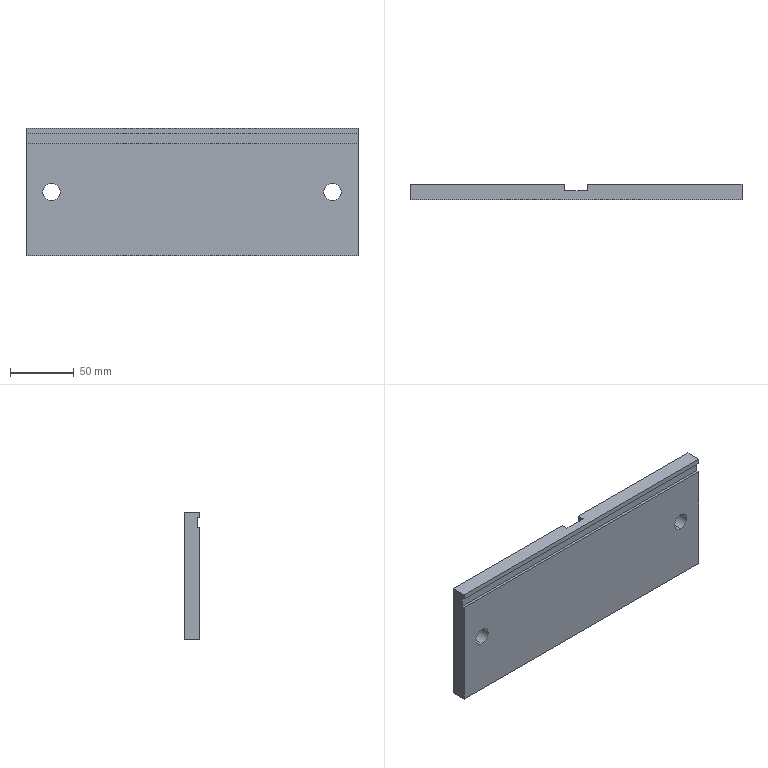Component | SolidWorks | NewTypeCurveBenderReducerPlate-DoubleWheel-2_NewCurveBender(New)ReducerBasePlate-DoubleWheel-1 | 1 solid | 18 faces | box 260 x 12 x 100 mm | volume 295405 mm3 | plane 14 | cylinder 4 | commonest cylinder face diameters 13.5 x4
build123d program:
from build123d import *

# Parameters (mm, degrees)
SKETCH1_W           = 260
SKETCH1_H           = 100
BOSS_EXTRUDE1_DEPTH = 12
SKETCH2_W           = 18
SKETCH2_H           = 5
CUT_EXTRUDE1_DEPTH  = 165.451
SKETCH3_R           = 6.75
CUT_EXTRUDE2_DEPTH  = 12
SKETCH5_W           = 8
SKETCH5_H           = 2
CUT_EXTRUDE3_DEPTH  = 266.036


with BuildPart() as part:
    # Sketch1 → Boss-Extrude1 (new body)
    with BuildSketch(Plane(origin=(0, 0, 0), x_dir=(1, 0, 0), z_dir=(0, 1, 0))):
        Rectangle(SKETCH1_W, SKETCH1_H)
    extrude(amount=BOSS_EXTRUDE1_DEPTH)

    # Sketch2 → Cut-Extrude1 (cut, through all)
    with BuildSketch(Plane.XY.offset(50)):
        with Locations((0, 2.5)):
            Rectangle(SKETCH2_W, SKETCH2_H)
    extrude(amount=-CUT_EXTRUDE1_DEPTH, mode=Mode.SUBTRACT)

    # Sketch3 → Cut-Extrude2 (cut)
    with BuildSketch(Plane(origin=(0, 12, 0), x_dir=(1, 0, 0), z_dir=(0, 1, 0))):
        with Locations(Location((-110, 0, 0), (0, 0, 270))):
            Circle(SKETCH3_R)
        with Locations(Location((110, 0, 0), (0, 0, 90))):
            Circle(SKETCH3_R)
    extrude(amount=-CUT_EXTRUDE2_DEPTH, mode=Mode.SUBTRACT)

    # Sketch5 → Cut-Extrude3 (cut, through all)
    with BuildSketch(Plane.ZY.offset(130)):
        with Locations((42, 11)):
            Rectangle(SKETCH5_W, SKETCH5_H)
    extrude(amount=-CUT_EXTRUDE3_DEPTH, mode=Mode.SUBTRACT)


solid = part.part

# Placed as in the assembly
solid = solid.moved(Location((0, 20, 158), (0, 0, 180)))
STEP:
#1=COLOUR_RGB('',0.7922,0.8196,0.9333);
#2=FILL_AREA_STYLE_COLOUR('',#1);
#3=FILL_AREA_STYLE('',(#2));
#4=SURFACE_STYLE_FILL_AREA(#3);
#5=SURFACE_SIDE_STYLE('',(#4));
#6=SURFACE_STYLE_USAGE(.BOTH.,#5);
#7=PRESENTATION_STYLE_ASSIGNMENT((#6));
#8=CARTESIAN_POINT('',(-4.331,0.7874,5.955));
#9=VERTEX_POINT('',#8);
#10=CARTESIAN_POINT('',(-4.331,0.7874,6.486));
#11=VERTEX_POINT('',#10);
#12=CARTESIAN_POINT('',(-4.331,0.7874,6.22));
#13=DIRECTION('',(-0.,-1.,-0.));
#14=DIRECTION('',(0.,0.,-1.));
#15=AXIS2_PLACEMENT_3D('',#12,#13,#14);
#16=CIRCLE('',#15,0.2657);
#17=EDGE_CURVE('',#9,#11,#16,.T.);
#18=ORIENTED_EDGE('',*,*,#17,.F.);
#19=CARTESIAN_POINT('',(-4.331,0.315,5.955));
#20=VERTEX_POINT('',#19);
#21=CARTESIAN_POINT('',(-4.331,0.7874,5.955));
#22=DIRECTION('',(-0.,-1.,-0.));
#23=VECTOR('',#22,39.37);
#24=LINE('',#21,#23);
#25=EDGE_CURVE('',#9,#20,#24,.T.);
#26=ORIENTED_EDGE('',*,*,#25,.T.);
#27=CARTESIAN_POINT('',(-4.331,0.315,6.486));
#28=VERTEX_POINT('',#27);
#29=CARTESIAN_POINT('',(-4.331,0.315,6.22));
#30=DIRECTION('',(-0.,-1.,-0.));
#31=DIRECTION('',(0.,0.,-1.));
#32=AXIS2_PLACEMENT_3D('',#29,#30,#31);
#33=CIRCLE('',#32,0.2657);
#34=EDGE_CURVE('',#20,#28,#33,.T.);
#35=ORIENTED_EDGE('',*,*,#34,.T.);
#36=CARTESIAN_POINT('',(-4.331,0.7874,6.486));
#37=DIRECTION('',(-0.,-1.,-0.));
#38=VECTOR('',#37,39.37);
#39=LINE('',#36,#38);
#40=EDGE_CURVE('',#11,#28,#39,.T.);
#41=ORIENTED_EDGE('',*,*,#40,.F.);
#42=EDGE_LOOP('',(#18,#26,#35,#41));
#43=FACE_OUTER_BOUND('',#42,.T.);
#44=CARTESIAN_POINT('',(-4.331,0.7874,6.22));
#45=DIRECTION('',(-0.,-1.,-0.));
#46=DIRECTION('',(0.,0.,1.));
#47=AXIS2_PLACEMENT_3D('',#44,#45,#46);
#48=CYLINDRICAL_SURFACE('',#47,0.2657);
#49=ADVANCED_FACE('',(#43),#48,.F.);
#50=CARTESIAN_POINT('',(4.331,0.7874,5.955));
#51=VERTEX_POINT('',#50);
#52=CARTESIAN_POINT('',(4.331,0.7874,6.486));
#53=VERTEX_POINT('',#52);
#54=CARTESIAN_POINT('',(4.331,0.7874,6.22));
#55=DIRECTION('',(-0.,-1.,-0.));
#56=DIRECTION('',(0.,0.,1.));
#57=AXIS2_PLACEMENT_3D('',#54,#55,#56);
#58=CIRCLE('',#57,0.2657);
#59=EDGE_CURVE('',#51,#53,#58,.T.);
#60=ORIENTED_EDGE('',*,*,#59,.F.);
#61=CARTESIAN_POINT('',(4.331,0.315,5.955));
#62=VERTEX_POINT('',#61);
#63=CARTESIAN_POINT('',(4.331,0.7874,5.955));
#64=DIRECTION('',(-0.,-1.,-0.));
#65=VECTOR('',#64,39.37);
#66=LINE('',#63,#65);
#67=EDGE_CURVE('',#51,#62,#66,.T.);
#68=ORIENTED_EDGE('',*,*,#67,.T.);
#69=CARTESIAN_POINT('',(4.331,0.315,6.486));
#70=VERTEX_POINT('',#69);
#71=CARTESIAN_POINT('',(4.331,0.315,6.22));
#72=DIRECTION('',(-0.,-1.,-0.));
#73=DIRECTION('',(0.,-0.,1.));
#74=AXIS2_PLACEMENT_3D('',#71,#72,#73);
#75=CIRCLE('',#74,0.2657);
#76=EDGE_CURVE('',#62,#70,#75,.T.);
#77=ORIENTED_EDGE('',*,*,#76,.T.);
#78=CARTESIAN_POINT('',(4.331,0.7874,6.486));
#79=DIRECTION('',(-0.,-1.,-0.));
#80=VECTOR('',#79,39.37);
#81=LINE('',#78,#80);
#82=EDGE_CURVE('',#53,#70,#81,.T.);
#83=ORIENTED_EDGE('',*,*,#82,.F.);
#84=EDGE_LOOP('',(#60,#68,#77,#83));
#85=FACE_OUTER_BOUND('',#84,.T.);
#86=CARTESIAN_POINT('',(4.331,0.7874,6.22));
#87=DIRECTION('',(-0.,-1.,-0.));
#88=DIRECTION('',(0.,0.,1.));
#89=AXIS2_PLACEMENT_3D('',#86,#87,#88);
#90=CYLINDRICAL_SURFACE('',#89,0.2657);
#91=ADVANCED_FACE('',(#85),#90,.F.);
#92=CARTESIAN_POINT('',(-5.118,0.315,7.717));
#93=VERTEX_POINT('',#92);
#94=CARTESIAN_POINT('',(5.118,0.315,7.717));
#95=VERTEX_POINT('',#94);
#96=CARTESIAN_POINT('',(-5.118,0.315,7.717));
#97=DIRECTION('',(1.,-0.,0.));
#98=VECTOR('',#97,39.37);
#99=LINE('',#96,#98);
#100=EDGE_CURVE('',#93,#95,#99,.T.);
#101=ORIENTED_EDGE('',*,*,#100,.F.);
#102=CARTESIAN_POINT('',(-5.118,0.315,4.252));
#103=VERTEX_POINT('',#102);
#104=CARTESIAN_POINT('',(-5.118,0.315,4.252));
#105=DIRECTION('',(0.,0.,-1.));
#106=VECTOR('',#105,39.37);
#107=LINE('',#104,#106);
#108=EDGE_CURVE('',#93,#103,#107,.T.);
#109=ORIENTED_EDGE('',*,*,#108,.T.);
#110=CARTESIAN_POINT('',(5.118,0.315,4.252));
#111=VERTEX_POINT('',#110);
#112=CARTESIAN_POINT('',(5.118,0.315,4.252));
#113=DIRECTION('',(1.,-0.,0.));
#114=VECTOR('',#113,39.37);
#115=LINE('',#112,#114);
#116=EDGE_CURVE('',#103,#111,#115,.T.);
#117=ORIENTED_EDGE('',*,*,#116,.T.);
#118=CARTESIAN_POINT('',(5.118,0.315,4.252));
#119=DIRECTION('',(-0.,-0.,1.));
#120=VECTOR('',#119,39.37);
#121=LINE('',#118,#120);
#122=EDGE_CURVE('',#111,#95,#121,.T.);
#123=ORIENTED_EDGE('',*,*,#122,.T.);
#124=EDGE_LOOP('',(#101,#109,#117,#123));
#125=FACE_OUTER_BOUND('',#124,.T.);
#126=CARTESIAN_POINT('',(4.331,0.315,6.22));
#127=DIRECTION('',(-0.,-1.,-0.));
#128=DIRECTION('',(0.,-0.,1.));
#129=AXIS2_PLACEMENT_3D('',#126,#127,#128);
#130=CIRCLE('',#129,0.2657);
#131=EDGE_CURVE('',#70,#62,#130,.T.);
#132=ORIENTED_EDGE('',*,*,#131,.F.);
#133=ORIENTED_EDGE('',*,*,#76,.F.);
#134=EDGE_LOOP('',(#132,#133));
#135=FACE_BOUND('',#134,.T.);
#136=CARTESIAN_POINT('',(-4.331,0.315,6.22));
#137=DIRECTION('',(-0.,-1.,-0.));
#138=DIRECTION('',(0.,0.,-1.));
#139=AXIS2_PLACEMENT_3D('',#136,#137,#138);
#140=CIRCLE('',#139,0.2657);
#141=EDGE_CURVE('',#28,#20,#140,.T.);
#142=ORIENTED_EDGE('',*,*,#141,.F.);
#143=ORIENTED_EDGE('',*,*,#34,.F.);
#144=EDGE_LOOP('',(#142,#143));
#145=FACE_BOUND('',#144,.T.);
#146=CARTESIAN_POINT('',(0.,0.315,6.22));
#147=DIRECTION('',(-0.,-1.,-0.));
#148=DIRECTION('',(-0.,-0.,1.));
#149=AXIS2_PLACEMENT_3D('',#146,#147,#148);
#150=PLANE('',#149);
#151=ADVANCED_FACE('',(#125,#135,#145),#150,.T.);
#152=CARTESIAN_POINT('',(-4.331,0.7874,6.22));
#153=DIRECTION('',(-0.,-1.,-0.));
#154=DIRECTION('',(0.,0.,-1.));
#155=AXIS2_PLACEMENT_3D('',#152,#153,#154);
#156=CIRCLE('',#155,0.2657);
#157=EDGE_CURVE('',#11,#9,#156,.T.);
#158=ORIENTED_EDGE('',*,*,#157,.T.);
#159=ORIENTED_EDGE('',*,*,#17,.T.);
#160=EDGE_LOOP('',(#158,#159));
#161=FACE_BOUND('',#160,.T.);
#162=CARTESIAN_POINT('',(-0.3543,0.7874,8.189));
#163=VERTEX_POINT('',#162);
#164=CARTESIAN_POINT('',(-5.118,0.7874,8.189));
#165=VERTEX_POINT('',#164);
#166=CARTESIAN_POINT('',(5.118,0.7874,8.189));
#167=DIRECTION('',(-1.,0.,-0.));
#168=VECTOR('',#167,39.37);
#169=LINE('',#166,#168);
#170=EDGE_CURVE('',#163,#165,#169,.T.);
#171=ORIENTED_EDGE('',*,*,#170,.F.);
#172=CARTESIAN_POINT('',(-0.3543,0.7874,4.252));
#173=VERTEX_POINT('',#172);
#174=CARTESIAN_POINT('',(-0.3543,0.7874,4.252));
#175=DIRECTION('',(-0.,-0.,1.));
#176=VECTOR('',#175,39.37);
#177=LINE('',#174,#176);
#178=EDGE_CURVE('',#173,#163,#177,.T.);
#179=ORIENTED_EDGE('',*,*,#178,.F.);
#180=CARTESIAN_POINT('',(-5.118,0.7874,4.252));
#181=VERTEX_POINT('',#180);
#182=CARTESIAN_POINT('',(5.118,0.7874,4.252));
#183=DIRECTION('',(1.,-0.,0.));
#184=VECTOR('',#183,39.37);
#185=LINE('',#182,#184);
#186=EDGE_CURVE('',#181,#173,#185,.T.);
#187=ORIENTED_EDGE('',*,*,#186,.F.);
#188=CARTESIAN_POINT('',(-5.118,0.7874,4.252));
#189=DIRECTION('',(0.,0.,-1.));
#190=VECTOR('',#189,39.37);
#191=LINE('',#188,#190);
#192=EDGE_CURVE('',#165,#181,#191,.T.);
#193=ORIENTED_EDGE('',*,*,#192,.F.);
#194=EDGE_LOOP('',(#171,#179,#187,#193));
#195=FACE_OUTER_BOUND('',#194,.T.);
#196=CARTESIAN_POINT('',(0.,0.7874,6.22));
#197=DIRECTION('',(-0.,-1.,-0.));
#198=DIRECTION('',(-0.,-0.,1.));
#199=AXIS2_PLACEMENT_3D('',#196,#197,#198);
#200=PLANE('',#199);
#201=ADVANCED_FACE('',(#161,#195),#200,.F.);
#202=ORIENTED_EDGE('',*,*,#108,.F.);
#203=CARTESIAN_POINT('',(-5.118,0.3937,7.717));
#204=VERTEX_POINT('',#203);
#205=CARTESIAN_POINT('',(-5.118,0.315,7.717));
#206=DIRECTION('',(0.,1.,0.));
#207=VECTOR('',#206,39.37);
#208=LINE('',#205,#207);
#209=EDGE_CURVE('',#93,#204,#208,.T.);
#210=ORIENTED_EDGE('',*,*,#209,.T.);
#211=CARTESIAN_POINT('',(-5.118,0.3937,8.031));
#212=VERTEX_POINT('',#211);
#213=CARTESIAN_POINT('',(-5.118,0.3937,7.717));
#214=DIRECTION('',(-0.,-0.,1.));
#215=VECTOR('',#214,39.37);
#216=LINE('',#213,#215);
#217=EDGE_CURVE('',#204,#212,#216,.T.);
#218=ORIENTED_EDGE('',*,*,#217,.T.);
#219=CARTESIAN_POINT('',(-5.118,0.315,8.031));
#220=VERTEX_POINT('',#219);
#221=CARTESIAN_POINT('',(-5.118,0.315,8.031));
#222=DIRECTION('',(-0.,-1.,-0.));
#223=VECTOR('',#222,39.37);
#224=LINE('',#221,#223);
#225=EDGE_CURVE('',#212,#220,#224,.T.);
#226=ORIENTED_EDGE('',*,*,#225,.T.);
#227=CARTESIAN_POINT('',(-5.118,0.315,8.189));
#228=VERTEX_POINT('',#227);
#229=CARTESIAN_POINT('',(-5.118,0.315,4.252));
#230=DIRECTION('',(0.,0.,-1.));
#231=VECTOR('',#230,39.37);
#232=LINE('',#229,#231);
#233=EDGE_CURVE('',#228,#220,#232,.T.);
#234=ORIENTED_EDGE('',*,*,#233,.F.);
#235=CARTESIAN_POINT('',(-5.118,0.315,8.189));
#236=DIRECTION('',(0.,1.,0.));
#237=VECTOR('',#236,39.37);
#238=LINE('',#235,#237);
#239=EDGE_CURVE('',#228,#165,#238,.T.);
#240=ORIENTED_EDGE('',*,*,#239,.T.);
#241=ORIENTED_EDGE('',*,*,#192,.T.);
#242=CARTESIAN_POINT('',(-5.118,0.315,4.252));
#243=DIRECTION('',(0.,1.,0.));
#244=VECTOR('',#243,39.37);
#245=LINE('',#242,#244);
#246=EDGE_CURVE('',#103,#181,#245,.T.);
#247=ORIENTED_EDGE('',*,*,#246,.F.);
#248=EDGE_LOOP('',(#202,#210,#218,#226,#234,#240,#241,#247));
#249=FACE_OUTER_BOUND('',#248,.T.);
#250=CARTESIAN_POINT('',(-5.118,0.315,4.252));
#251=DIRECTION('',(1.,-0.,0.));
#252=DIRECTION('',(-0.,-0.,1.));
#253=AXIS2_PLACEMENT_3D('',#250,#251,#252);
#254=PLANE('',#253);
#255=ADVANCED_FACE('',(#249),#254,.F.);
#256=ORIENTED_EDGE('',*,*,#186,.T.);
#257=CARTESIAN_POINT('',(-0.3543,0.5906,4.252));
#258=VERTEX_POINT('',#257);
#259=CARTESIAN_POINT('',(-0.3543,0.7874,4.252));
#260=DIRECTION('',(-0.,-1.,-0.));
#261=VECTOR('',#260,39.37);
#262=LINE('',#259,#261);
#263=EDGE_CURVE('',#173,#258,#262,.T.);
#264=ORIENTED_EDGE('',*,*,#263,.T.);
#265=CARTESIAN_POINT('',(0.3543,0.5906,4.252));
#266=VERTEX_POINT('',#265);
#267=CARTESIAN_POINT('',(-0.3543,0.5906,4.252));
#268=DIRECTION('',(1.,0.,0.));
#269=VECTOR('',#268,39.37);
#270=LINE('',#267,#269);
#271=EDGE_CURVE('',#258,#266,#270,.T.);
#272=ORIENTED_EDGE('',*,*,#271,.T.);
#273=CARTESIAN_POINT('',(0.3543,0.7874,4.252));
#274=VERTEX_POINT('',#273);
#275=CARTESIAN_POINT('',(0.3543,0.7874,4.252));
#276=DIRECTION('',(0.,1.,0.));
#277=VECTOR('',#276,39.37);
#278=LINE('',#275,#277);
#279=EDGE_CURVE('',#266,#274,#278,.T.);
#280=ORIENTED_EDGE('',*,*,#279,.T.);
#281=CARTESIAN_POINT('',(5.118,0.7874,4.252));
#282=VERTEX_POINT('',#281);
#283=CARTESIAN_POINT('',(5.118,0.7874,4.252));
#284=DIRECTION('',(1.,-0.,0.));
#285=VECTOR('',#284,39.37);
#286=LINE('',#283,#285);
#287=EDGE_CURVE('',#274,#282,#286,.T.);
#288=ORIENTED_EDGE('',*,*,#287,.T.);
#289=CARTESIAN_POINT('',(5.118,0.315,4.252));
#290=DIRECTION('',(0.,1.,0.));
#291=VECTOR('',#290,39.37);
#292=LINE('',#289,#291);
#293=EDGE_CURVE('',#111,#282,#292,.T.);
#294=ORIENTED_EDGE('',*,*,#293,.F.);
#295=ORIENTED_EDGE('',*,*,#116,.F.);
#296=ORIENTED_EDGE('',*,*,#246,.T.);
#297=EDGE_LOOP('',(#256,#264,#272,#280,#288,#294,#295,#296));
#298=FACE_OUTER_BOUND('',#297,.T.);
#299=CARTESIAN_POINT('',(5.118,0.315,4.252));
#300=DIRECTION('',(-0.,-0.,1.));
#301=DIRECTION('',(-1.,0.,-0.));
#302=AXIS2_PLACEMENT_3D('',#299,#300,#301);
#303=PLANE('',#302);
#304=ADVANCED_FACE('',(#298),#303,.F.);
#305=CARTESIAN_POINT('',(5.118,0.3937,7.717));
#306=VERTEX_POINT('',#305);
#307=CARTESIAN_POINT('',(5.118,0.3937,8.031));
#308=VERTEX_POINT('',#307);
#309=CARTESIAN_POINT('',(5.118,0.3937,7.717));
#310=DIRECTION('',(-0.,-0.,1.));
#311=VECTOR('',#310,39.37);
#312=LINE('',#309,#311);
#313=EDGE_CURVE('',#306,#308,#312,.T.);
#314=ORIENTED_EDGE('',*,*,#313,.F.);
#315=CARTESIAN_POINT('',(5.118,0.315,7.717));
#316=DIRECTION('',(0.,1.,0.));
#317=VECTOR('',#316,39.37);
#318=LINE('',#315,#317);
#319=EDGE_CURVE('',#95,#306,#318,.T.);
#320=ORIENTED_EDGE('',*,*,#319,.F.);
#321=ORIENTED_EDGE('',*,*,#122,.F.);
#322=ORIENTED_EDGE('',*,*,#293,.T.);
#323=CARTESIAN_POINT('',(5.118,0.7874,8.189));
#324=VERTEX_POINT('',#323);
#325=CARTESIAN_POINT('',(5.118,0.7874,4.252));
#326=DIRECTION('',(-0.,-0.,1.));
#327=VECTOR('',#326,39.37);
#328=LINE('',#325,#327);
#329=EDGE_CURVE('',#282,#324,#328,.T.);
#330=ORIENTED_EDGE('',*,*,#329,.T.);
#331=CARTESIAN_POINT('',(5.118,0.315,8.189));
#332=VERTEX_POINT('',#331);
#333=CARTESIAN_POINT('',(5.118,0.315,8.189));
#334=DIRECTION('',(0.,1.,0.));
#335=VECTOR('',#334,39.37);
#336=LINE('',#333,#335);
#337=EDGE_CURVE('',#332,#324,#336,.T.);
#338=ORIENTED_EDGE('',*,*,#337,.F.);
#339=CARTESIAN_POINT('',(5.118,0.315,8.031));
#340=VERTEX_POINT('',#339);
#341=CARTESIAN_POINT('',(5.118,0.315,4.252));
#342=DIRECTION('',(-0.,-0.,1.));
#343=VECTOR('',#342,39.37);
#344=LINE('',#341,#343);
#345=EDGE_CURVE('',#340,#332,#344,.T.);
#346=ORIENTED_EDGE('',*,*,#345,.F.);
#347=CARTESIAN_POINT('',(5.118,0.315,8.031));
#348=DIRECTION('',(-0.,-1.,-0.));
#349=VECTOR('',#348,39.37);
#350=LINE('',#347,#349);
#351=EDGE_CURVE('',#308,#340,#350,.T.);
#352=ORIENTED_EDGE('',*,*,#351,.F.);
#353=EDGE_LOOP('',(#314,#320,#321,#322,#330,#338,#346,#352));
#354=FACE_OUTER_BOUND('',#353,.T.);
#355=CARTESIAN_POINT('',(5.118,0.315,4.252));
#356=DIRECTION('',(-1.,0.,-0.));
#357=DIRECTION('',(0.,0.,-1.));
#358=AXIS2_PLACEMENT_3D('',#355,#356,#357);
#359=PLANE('',#358);
#360=ADVANCED_FACE('',(#354),#359,.F.);
#361=CARTESIAN_POINT('',(-0.3543,0.5906,8.189));
#362=VERTEX_POINT('',#361);
#363=CARTESIAN_POINT('',(0.3543,0.5906,8.189));
#364=VERTEX_POINT('',#363);
#365=CARTESIAN_POINT('',(-0.3543,0.5906,8.189));
#366=DIRECTION('',(1.,0.,0.));
#367=VECTOR('',#366,39.37);
#368=LINE('',#365,#367);
#369=EDGE_CURVE('',#362,#364,#368,.T.);
#370=ORIENTED_EDGE('',*,*,#369,.F.);
#371=CARTESIAN_POINT('',(-0.3543,0.7874,8.189));
#372=DIRECTION('',(-0.,-1.,-0.));
#373=VECTOR('',#372,39.37);
#374=LINE('',#371,#373);
#375=EDGE_CURVE('',#163,#362,#374,.T.);
#376=ORIENTED_EDGE('',*,*,#375,.F.);
#377=ORIENTED_EDGE('',*,*,#170,.T.);
#378=ORIENTED_EDGE('',*,*,#239,.F.);
#379=CARTESIAN_POINT('',(5.118,0.315,8.189));
#380=DIRECTION('',(-1.,0.,-0.));
#381=VECTOR('',#380,39.37);
#382=LINE('',#379,#381);
#383=EDGE_CURVE('',#332,#228,#382,.T.);
#384=ORIENTED_EDGE('',*,*,#383,.F.);
#385=ORIENTED_EDGE('',*,*,#337,.T.);
#386=CARTESIAN_POINT('',(0.3543,0.7874,8.189));
#387=VERTEX_POINT('',#386);
#388=CARTESIAN_POINT('',(5.118,0.7874,8.189));
#389=DIRECTION('',(-1.,0.,-0.));
#390=VECTOR('',#389,39.37);
#391=LINE('',#388,#390);
#392=EDGE_CURVE('',#324,#387,#391,.T.);
#393=ORIENTED_EDGE('',*,*,#392,.T.);
#394=CARTESIAN_POINT('',(0.3543,0.7874,8.189));
#395=DIRECTION('',(0.,1.,0.));
#396=VECTOR('',#395,39.37);
#397=LINE('',#394,#396);
#398=EDGE_CURVE('',#364,#387,#397,.T.);
#399=ORIENTED_EDGE('',*,*,#398,.F.);
#400=EDGE_LOOP('',(#370,#376,#377,#378,#384,#385,#393,#399));
#401=FACE_OUTER_BOUND('',#400,.T.);
#402=CARTESIAN_POINT('',(5.118,0.315,8.189));
#403=DIRECTION('',(0.,0.,-1.));
#404=DIRECTION('',(1.,-0.,0.));
#405=AXIS2_PLACEMENT_3D('',#402,#403,#404);
#406=PLANE('',#405);
#407=ADVANCED_FACE('',(#401),#406,.F.);
#408=CARTESIAN_POINT('',(-5.118,0.315,8.031));
#409=DIRECTION('',(1.,-0.,0.));
#410=VECTOR('',#409,39.37);
#411=LINE('',#408,#410);
#412=EDGE_CURVE('',#220,#340,#411,.T.);
#413=ORIENTED_EDGE('',*,*,#412,.T.);
#414=ORIENTED_EDGE('',*,*,#345,.T.);
#415=ORIENTED_EDGE('',*,*,#383,.T.);
#416=ORIENTED_EDGE('',*,*,#233,.T.);
#417=EDGE_LOOP('',(#413,#414,#415,#416));
#418=FACE_OUTER_BOUND('',#417,.T.);
#419=CARTESIAN_POINT('',(0.,0.315,6.22));
#420=DIRECTION('',(-0.,-1.,-0.));
#421=DIRECTION('',(-0.,-0.,1.));
#422=AXIS2_PLACEMENT_3D('',#419,#420,#421);
#423=PLANE('',#422);
#424=ADVANCED_FACE('',(#418),#423,.T.);
#425=CARTESIAN_POINT('',(4.331,0.7874,6.22));
#426=DIRECTION('',(-0.,-1.,-0.));
#427=DIRECTION('',(0.,0.,1.));
#428=AXIS2_PLACEMENT_3D('',#425,#426,#427);
#429=CIRCLE('',#428,0.2657);
#430=EDGE_CURVE('',#53,#51,#429,.T.);
#431=ORIENTED_EDGE('',*,*,#430,.T.);
#432=ORIENTED_EDGE('',*,*,#59,.T.);
#433=EDGE_LOOP('',(#431,#432));
#434=FACE_BOUND('',#433,.T.);
#435=ORIENTED_EDGE('',*,*,#287,.F.);
#436=CARTESIAN_POINT('',(0.3543,0.7874,4.252));
#437=DIRECTION('',(-0.,-0.,1.));
#438=VECTOR('',#437,39.37);
#439=LINE('',#436,#438);
#440=EDGE_CURVE('',#274,#387,#439,.T.);
#441=ORIENTED_EDGE('',*,*,#440,.T.);
#442=ORIENTED_EDGE('',*,*,#392,.F.);
#443=ORIENTED_EDGE('',*,*,#329,.F.);
#444=EDGE_LOOP('',(#435,#441,#442,#443));
#445=FACE_OUTER_BOUND('',#444,.T.);
#446=CARTESIAN_POINT('',(0.,0.7874,6.22));
#447=DIRECTION('',(-0.,-1.,-0.));
#448=DIRECTION('',(-0.,-0.,1.));
#449=AXIS2_PLACEMENT_3D('',#446,#447,#448);
#450=PLANE('',#449);
#451=ADVANCED_FACE('',(#434,#445),#450,.F.);
#452=ORIENTED_EDGE('',*,*,#375,.T.);
#453=CARTESIAN_POINT('',(-0.3543,0.5906,4.252));
#454=DIRECTION('',(-0.,-0.,1.));
#455=VECTOR('',#454,39.37);
#456=LINE('',#453,#455);
#457=EDGE_CURVE('',#258,#362,#456,.T.);
#458=ORIENTED_EDGE('',*,*,#457,.F.);
#459=ORIENTED_EDGE('',*,*,#263,.F.);
#460=ORIENTED_EDGE('',*,*,#178,.T.);
#461=EDGE_LOOP('',(#452,#458,#459,#460));
#462=FACE_OUTER_BOUND('',#461,.T.);
#463=CARTESIAN_POINT('',(-0.3543,0.7874,4.252));
#464=DIRECTION('',(-1.,0.,-0.));
#465=DIRECTION('',(0.,0.,-1.));
#466=AXIS2_PLACEMENT_3D('',#463,#464,#465);
#467=PLANE('',#466);
#468=ADVANCED_FACE('',(#462),#467,.F.);
#469=ORIENTED_EDGE('',*,*,#398,.T.);
#470=ORIENTED_EDGE('',*,*,#440,.F.);
#471=ORIENTED_EDGE('',*,*,#279,.F.);
#472=CARTESIAN_POINT('',(0.3543,0.5906,4.252));
#473=DIRECTION('',(-0.,-0.,1.));
#474=VECTOR('',#473,39.37);
#475=LINE('',#472,#474);
#476=EDGE_CURVE('',#266,#364,#475,.T.);
#477=ORIENTED_EDGE('',*,*,#476,.T.);
#478=EDGE_LOOP('',(#469,#470,#471,#477));
#479=FACE_OUTER_BOUND('',#478,.T.);
#480=CARTESIAN_POINT('',(0.3543,0.7874,4.252));
#481=DIRECTION('',(1.,-0.,0.));
#482=DIRECTION('',(-0.,-0.,1.));
#483=AXIS2_PLACEMENT_3D('',#480,#481,#482);
#484=PLANE('',#483);
#485=ADVANCED_FACE('',(#479),#484,.F.);
#486=ORIENTED_EDGE('',*,*,#369,.T.);
#487=ORIENTED_EDGE('',*,*,#476,.F.);
#488=ORIENTED_EDGE('',*,*,#271,.F.);
#489=ORIENTED_EDGE('',*,*,#457,.T.);
#490=EDGE_LOOP('',(#486,#487,#488,#489));
#491=FACE_OUTER_BOUND('',#490,.T.);
#492=CARTESIAN_POINT('',(-0.3543,0.5906,4.252));
#493=DIRECTION('',(0.,-1.,-0.));
#494=DIRECTION('',(1.,0.,0.));
#495=AXIS2_PLACEMENT_3D('',#492,#493,#494);
#496=PLANE('',#495);
#497=ADVANCED_FACE('',(#491),#496,.F.);
#498=ORIENTED_EDGE('',*,*,#67,.F.);
#499=ORIENTED_EDGE('',*,*,#430,.F.);
#500=ORIENTED_EDGE('',*,*,#82,.T.);
#501=ORIENTED_EDGE('',*,*,#131,.T.);
#502=EDGE_LOOP('',(#498,#499,#500,#501));
#503=FACE_OUTER_BOUND('',#502,.T.);
#504=CARTESIAN_POINT('',(4.331,0.7874,6.22));
#505=DIRECTION('',(-0.,-1.,-0.));
#506=DIRECTION('',(0.,0.,1.));
#507=AXIS2_PLACEMENT_3D('',#504,#505,#506);
#508=CYLINDRICAL_SURFACE('',#507,0.2657);
#509=ADVANCED_FACE('',(#503),#508,.F.);
#510=ORIENTED_EDGE('',*,*,#25,.F.);
#511=ORIENTED_EDGE('',*,*,#157,.F.);
#512=ORIENTED_EDGE('',*,*,#40,.T.);
#513=ORIENTED_EDGE('',*,*,#141,.T.);
#514=EDGE_LOOP('',(#510,#511,#512,#513));
#515=FACE_OUTER_BOUND('',#514,.T.);
#516=CARTESIAN_POINT('',(-4.331,0.7874,6.22));
#517=DIRECTION('',(-0.,-1.,-0.));
#518=DIRECTION('',(0.,0.,1.));
#519=AXIS2_PLACEMENT_3D('',#516,#517,#518);
#520=CYLINDRICAL_SURFACE('',#519,0.2657);
#521=ADVANCED_FACE('',(#515),#520,.F.);
#522=ORIENTED_EDGE('',*,*,#319,.T.);
#523=CARTESIAN_POINT('',(-5.118,0.3937,7.717));
#524=DIRECTION('',(1.,-0.,0.));
#525=VECTOR('',#524,39.37);
#526=LINE('',#523,#525);
#527=EDGE_CURVE('',#204,#306,#526,.T.);
#528=ORIENTED_EDGE('',*,*,#527,.F.);
#529=ORIENTED_EDGE('',*,*,#209,.F.);
#530=ORIENTED_EDGE('',*,*,#100,.T.);
#531=EDGE_LOOP('',(#522,#528,#529,#530));
#532=FACE_OUTER_BOUND('',#531,.T.);
#533=CARTESIAN_POINT('',(-5.118,0.315,7.717));
#534=DIRECTION('',(0.,0.,-1.));
#535=DIRECTION('',(1.,-0.,0.));
#536=AXIS2_PLACEMENT_3D('',#533,#534,#535);
#537=PLANE('',#536);
#538=ADVANCED_FACE('',(#532),#537,.F.);
#539=ORIENTED_EDGE('',*,*,#351,.T.);
#540=ORIENTED_EDGE('',*,*,#412,.F.);
#541=ORIENTED_EDGE('',*,*,#225,.F.);
#542=CARTESIAN_POINT('',(-5.118,0.3937,8.031));
#543=DIRECTION('',(1.,-0.,0.));
#544=VECTOR('',#543,39.37);
#545=LINE('',#542,#544);
#546=EDGE_CURVE('',#212,#308,#545,.T.);
#547=ORIENTED_EDGE('',*,*,#546,.T.);
#548=EDGE_LOOP('',(#539,#540,#541,#547));
#549=FACE_OUTER_BOUND('',#548,.T.);
#550=CARTESIAN_POINT('',(-5.118,0.315,8.031));
#551=DIRECTION('',(-0.,-0.,1.));
#552=DIRECTION('',(-1.,0.,-0.));
#553=AXIS2_PLACEMENT_3D('',#550,#551,#552);
#554=PLANE('',#553);
#555=ADVANCED_FACE('',(#549),#554,.F.);
#556=ORIENTED_EDGE('',*,*,#313,.T.);
#557=ORIENTED_EDGE('',*,*,#546,.F.);
#558=ORIENTED_EDGE('',*,*,#217,.F.);
#559=ORIENTED_EDGE('',*,*,#527,.T.);
#560=EDGE_LOOP('',(#556,#557,#558,#559));
#561=FACE_OUTER_BOUND('',#560,.T.);
#562=CARTESIAN_POINT('',(-5.118,0.3937,7.717));
#563=DIRECTION('',(0.,1.,0.));
#564=DIRECTION('',(0.,0.,-1.));
#565=AXIS2_PLACEMENT_3D('',#562,#563,#564);
#566=PLANE('',#565);
#567=ADVANCED_FACE('',(#561),#566,.F.);
#568=CLOSED_SHELL('',(#49,#91,#151,#201,#255,#304,#360,#407,#424,#451,#468,#485,#497,#509,#521,#538,#555,#567));
#569=MANIFOLD_SOLID_BREP('',#568);
#570=STYLED_ITEM('',(#7),#569);
#571=(LENGTH_UNIT()NAMED_UNIT(*)SI_UNIT($,.METRE.));
#572=LENGTH_MEASURE_WITH_UNIT(LENGTH_MEASURE(0.0254),#571);
#573=DIMENSIONAL_EXPONENTS(1.,0.,0.,0.,0.,0.,0.);
#574=(CONVERSION_BASED_UNIT('',#572)LENGTH_UNIT()NAMED_UNIT(#573));
#575=UNCERTAINTY_MEASURE_WITH_UNIT(LENGTH_MEASURE(0.00001),#574,'','');
#576=(NAMED_UNIT(*)PLANE_ANGLE_UNIT()SI_UNIT($,.RADIAN.));
#577=(NAMED_UNIT(*)SI_UNIT($,.STERADIAN.)SOLID_ANGLE_UNIT());
#578=(GEOMETRIC_REPRESENTATION_CONTEXT(3)GLOBAL_UNCERTAINTY_ASSIGNED_CONTEXT((#575))GLOBAL_UNIT_ASSIGNED_CONTEXT((#574,#576,#577))REPRESENTATION_CONTEXT('',''));
#579=MECHANICAL_DESIGN_GEOMETRIC_PRESENTATION_REPRESENTATION('',(#570),#578);
#580=PRESENTATION_LAYER_ASSIGNMENT('','',(#570));
#581=CARTESIAN_POINT('',(0.,0.,0.));
#582=DIRECTION('',(0.,0.,1.));
#583=DIRECTION('',(1.,0.,0.));
#584=AXIS2_PLACEMENT_3D('',#581,#582,#583);
#585=(LENGTH_UNIT()NAMED_UNIT(*)SI_UNIT($,.METRE.));
#586=LENGTH_MEASURE_WITH_UNIT(LENGTH_MEASURE(0.0254),#585);
#587=DIMENSIONAL_EXPONENTS(1.,0.,0.,0.,0.,0.,0.);
#588=(CONVERSION_BASED_UNIT('',#586)LENGTH_UNIT()NAMED_UNIT(#587));
#589=UNCERTAINTY_MEASURE_WITH_UNIT(LENGTH_MEASURE(0.00001),#588,'','');
#590=(NAMED_UNIT(*)PLANE_ANGLE_UNIT()SI_UNIT($,.RADIAN.));
#591=(NAMED_UNIT(*)SI_UNIT($,.STERADIAN.)SOLID_ANGLE_UNIT());
#592=(GEOMETRIC_REPRESENTATION_CONTEXT(3)GLOBAL_UNCERTAINTY_ASSIGNED_CONTEXT((#589))GLOBAL_UNIT_ASSIGNED_CONTEXT((#588,#590,#591))REPRESENTATION_CONTEXT('',''));
#593=ADVANCED_BREP_SHAPE_REPRESENTATION('',(#569,#584),#592);